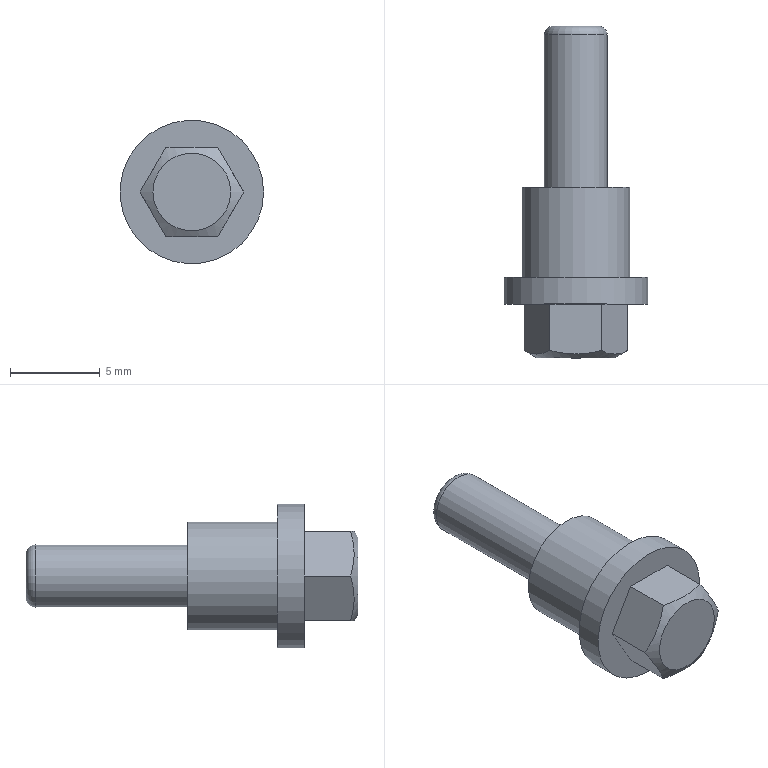Component | NX | OUTER_CASING_TUBE_SMALL_BOLT | 1 solid | 16 faces | volume 367 mm3 | plane 11 | cylinder 3 | cone 1 | torus 1 | commonest cylinder face diameters 3.5 x1 6 x1 8 x1